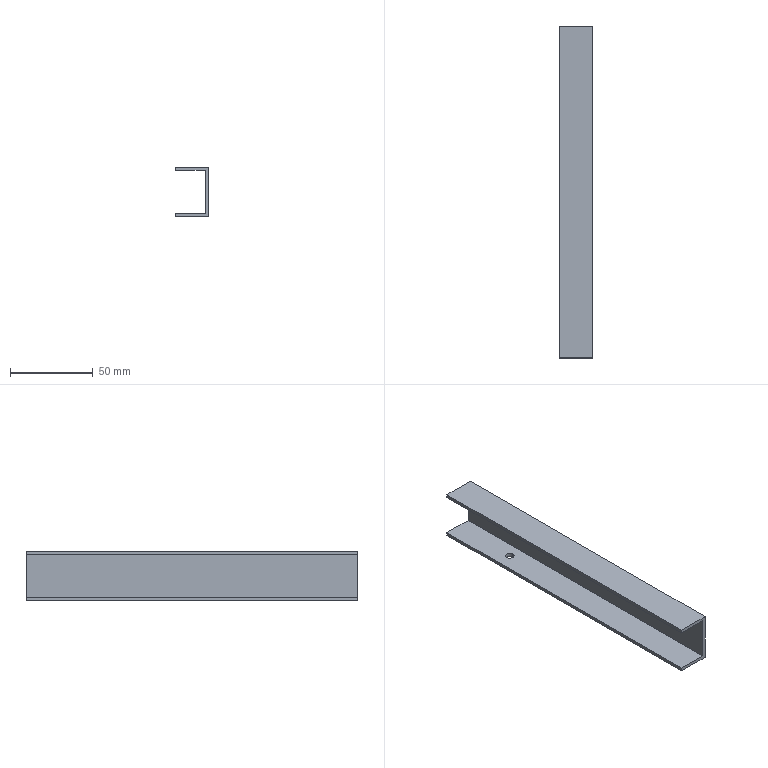Component | SolidWorks | Copy_of_Copy_of_Part4-1 | 1 solid | 12 faces | box 20 x 200 x 30 mm | volume 26361 mm3 | plane 10 | cylinder 2 | commonest cylinder face diameters 5 x2
build123d program:
from build123d import *

# Parameters (mm, degrees)
EXTRUDE_THIN1_DEPTH = 200
SKETCH4_R           = 2.5
CUT_EXTRUDE1_DEPTH  = 10


with BuildPart() as part:
    # Sketch2 → Extrude-Thin1 (new body)
    with BuildSketch(Plane(origin=(0, 0, 0), x_dir=(1, 0, 0), z_dir=(0, 1, 0))):
        Polygon((-173.819, 20), (-173.819, 0), (-143.819, 0), (-143.819, 20), (-145.819, 20), (-145.819, 2), (-171.819, 2), (-171.819, 20), align=None)
    extrude(amount=EXTRUDE_THIN1_DEPTH)

    # Sketch4 → Cut-Extrude1 (cut)
    with BuildSketch(Plane(origin=(-143.819, 0, 0), x_dir=(0, 0, -1), z_dir=(1, 0, 0))):
        with Locations((10.231, 156.085)):
            Circle(SKETCH4_R)
    extrude(amount=-CUT_EXTRUDE1_DEPTH, mode=Mode.SUBTRACT)


solid = part.part

# Placed as in the assembly
solid = solid.moved(Location((152, 30, -459.911), (0, 90, 0)))
STEP:
#1=CARTESIAN_POINT('',(5.68,7.326,-12.366));
#2=VERTEX_POINT('',#1);
#3=CARTESIAN_POINT('',(5.483,7.326,-12.366));
#4=VERTEX_POINT('',#3);
#5=CARTESIAN_POINT('',(5.581,7.326,-12.366));
#6=DIRECTION('',(0.,0.,-1.));
#7=DIRECTION('',(-1.,0.,0.));
#8=AXIS2_PLACEMENT_3D('',#5,#6,#7);
#9=CIRCLE('',#8,0.09843);
#10=EDGE_CURVE('',#2,#4,#9,.T.);
#11=ORIENTED_EDGE('',*,*,#10,.F.);
#12=CARTESIAN_POINT('',(5.68,7.326,-12.445));
#13=VERTEX_POINT('',#12);
#14=CARTESIAN_POINT('',(5.68,7.326,-12.051));
#15=DIRECTION('',(0.,0.,-1.));
#16=VECTOR('',#15,39.37);
#17=LINE('',#14,#16);
#18=EDGE_CURVE('',#2,#13,#17,.T.);
#19=ORIENTED_EDGE('',*,*,#18,.T.);
#20=CARTESIAN_POINT('',(5.483,7.326,-12.445));
#21=VERTEX_POINT('',#20);
#22=CARTESIAN_POINT('',(5.581,7.326,-12.445));
#23=DIRECTION('',(0.,0.,-1.));
#24=DIRECTION('',(-1.,0.,0.));
#25=AXIS2_PLACEMENT_3D('',#22,#23,#24);
#26=CIRCLE('',#25,0.09843);
#27=EDGE_CURVE('',#13,#21,#26,.T.);
#28=ORIENTED_EDGE('',*,*,#27,.T.);
#29=CARTESIAN_POINT('',(5.483,7.326,-12.051));
#30=DIRECTION('',(0.,0.,-1.));
#31=VECTOR('',#30,39.37);
#32=LINE('',#29,#31);
#33=EDGE_CURVE('',#4,#21,#32,.T.);
#34=ORIENTED_EDGE('',*,*,#33,.F.);
#35=EDGE_LOOP('',(#11,#19,#28,#34));
#36=FACE_OUTER_BOUND('',#35,.T.);
#37=CARTESIAN_POINT('',(5.581,7.326,-12.051));
#38=DIRECTION('',(0.,0.,-1.));
#39=DIRECTION('',(-1.,0.,0.));
#40=AXIS2_PLACEMENT_3D('',#37,#38,#39);
#41=CYLINDRICAL_SURFACE('',#40,0.09843);
#42=ADVANCED_FACE('',(#36),#41,.F.);
#43=CARTESIAN_POINT('',(5.906,1.181,-11.342));
#44=VERTEX_POINT('',#43);
#45=CARTESIAN_POINT('',(5.197,1.181,-11.342));
#46=VERTEX_POINT('',#45);
#47=CARTESIAN_POINT('',(5.197,1.181,-11.342));
#48=DIRECTION('',(-1.,0.,0.));
#49=VECTOR('',#48,39.37);
#50=LINE('',#47,#49);
#51=EDGE_CURVE('',#44,#46,#50,.T.);
#52=ORIENTED_EDGE('',*,*,#51,.T.);
#53=CARTESIAN_POINT('',(5.197,9.055,-11.342));
#54=VERTEX_POINT('',#53);
#55=CARTESIAN_POINT('',(5.197,9.055,-11.342));
#56=DIRECTION('',(0.,-1.,0.));
#57=VECTOR('',#56,39.37);
#58=LINE('',#55,#57);
#59=EDGE_CURVE('',#54,#46,#58,.T.);
#60=ORIENTED_EDGE('',*,*,#59,.F.);
#61=CARTESIAN_POINT('',(5.906,9.055,-11.342));
#62=VERTEX_POINT('',#61);
#63=CARTESIAN_POINT('',(5.197,9.055,-11.342));
#64=DIRECTION('',(-1.,0.,0.));
#65=VECTOR('',#64,39.37);
#66=LINE('',#63,#65);
#67=EDGE_CURVE('',#62,#54,#66,.T.);
#68=ORIENTED_EDGE('',*,*,#67,.F.);
#69=CARTESIAN_POINT('',(5.906,9.055,-11.342));
#70=DIRECTION('',(0.,-1.,0.));
#71=VECTOR('',#70,39.37);
#72=LINE('',#69,#71);
#73=EDGE_CURVE('',#62,#44,#72,.T.);
#74=ORIENTED_EDGE('',*,*,#73,.T.);
#75=EDGE_LOOP('',(#52,#60,#68,#74));
#76=FACE_OUTER_BOUND('',#75,.T.);
#77=CARTESIAN_POINT('',(5.197,9.055,-11.342));
#78=DIRECTION('',(0.,0.,1.));
#79=DIRECTION('',(1.,0.,0.));
#80=AXIS2_PLACEMENT_3D('',#77,#78,#79);
#81=PLANE('',#80);
#82=ADVANCED_FACE('',(#76),#81,.F.);
#83=CARTESIAN_POINT('',(5.197,1.181,-11.263));
#84=VERTEX_POINT('',#83);
#85=CARTESIAN_POINT('',(5.197,1.181,-11.263));
#86=DIRECTION('',(0.,0.,-1.));
#87=VECTOR('',#86,39.37);
#88=LINE('',#85,#87);
#89=EDGE_CURVE('',#84,#46,#88,.T.);
#90=ORIENTED_EDGE('',*,*,#89,.F.);
#91=CARTESIAN_POINT('',(5.197,9.055,-11.263));
#92=VERTEX_POINT('',#91);
#93=CARTESIAN_POINT('',(5.197,9.055,-11.263));
#94=DIRECTION('',(0.,-1.,0.));
#95=VECTOR('',#94,39.37);
#96=LINE('',#93,#95);
#97=EDGE_CURVE('',#92,#84,#96,.T.);
#98=ORIENTED_EDGE('',*,*,#97,.F.);
#99=CARTESIAN_POINT('',(5.197,9.055,-11.263));
#100=DIRECTION('',(0.,0.,-1.));
#101=VECTOR('',#100,39.37);
#102=LINE('',#99,#101);
#103=EDGE_CURVE('',#92,#54,#102,.T.);
#104=ORIENTED_EDGE('',*,*,#103,.T.);
#105=ORIENTED_EDGE('',*,*,#59,.T.);
#106=EDGE_LOOP('',(#90,#98,#104,#105));
#107=FACE_OUTER_BOUND('',#106,.T.);
#108=CARTESIAN_POINT('',(5.197,9.055,-11.263));
#109=DIRECTION('',(-1.,0.,0.));
#110=DIRECTION('',(0.,0.,1.));
#111=AXIS2_PLACEMENT_3D('',#108,#109,#110);
#112=PLANE('',#111);
#113=ADVANCED_FACE('',(#107),#112,.T.);
#114=CARTESIAN_POINT('',(5.984,1.181,-11.263));
#115=VERTEX_POINT('',#114);
#116=CARTESIAN_POINT('',(5.197,1.181,-11.263));
#117=DIRECTION('',(-1.,0.,0.));
#118=VECTOR('',#117,39.37);
#119=LINE('',#116,#118);
#120=EDGE_CURVE('',#115,#84,#119,.T.);
#121=ORIENTED_EDGE('',*,*,#120,.F.);
#122=CARTESIAN_POINT('',(5.984,9.055,-11.263));
#123=VERTEX_POINT('',#122);
#124=CARTESIAN_POINT('',(5.984,9.055,-11.263));
#125=DIRECTION('',(0.,-1.,0.));
#126=VECTOR('',#125,39.37);
#127=LINE('',#124,#126);
#128=EDGE_CURVE('',#123,#115,#127,.T.);
#129=ORIENTED_EDGE('',*,*,#128,.F.);
#130=CARTESIAN_POINT('',(5.197,9.055,-11.263));
#131=DIRECTION('',(-1.,0.,0.));
#132=VECTOR('',#131,39.37);
#133=LINE('',#130,#132);
#134=EDGE_CURVE('',#123,#92,#133,.T.);
#135=ORIENTED_EDGE('',*,*,#134,.T.);
#136=ORIENTED_EDGE('',*,*,#97,.T.);
#137=EDGE_LOOP('',(#121,#129,#135,#136));
#138=FACE_OUTER_BOUND('',#137,.T.);
#139=CARTESIAN_POINT('',(5.197,9.055,-11.263));
#140=DIRECTION('',(0.,0.,1.));
#141=DIRECTION('',(1.,0.,0.));
#142=AXIS2_PLACEMENT_3D('',#139,#140,#141);
#143=PLANE('',#142);
#144=ADVANCED_FACE('',(#138),#143,.T.);
#145=CARTESIAN_POINT('',(5.984,1.181,-12.445));
#146=VERTEX_POINT('',#145);
#147=CARTESIAN_POINT('',(5.984,1.181,-11.263));
#148=DIRECTION('',(0.,0.,1.));
#149=VECTOR('',#148,39.37);
#150=LINE('',#147,#149);
#151=EDGE_CURVE('',#146,#115,#150,.T.);
#152=ORIENTED_EDGE('',*,*,#151,.F.);
#153=CARTESIAN_POINT('',(5.984,9.055,-12.445));
#154=VERTEX_POINT('',#153);
#155=CARTESIAN_POINT('',(5.984,9.055,-12.445));
#156=DIRECTION('',(0.,-1.,0.));
#157=VECTOR('',#156,39.37);
#158=LINE('',#155,#157);
#159=EDGE_CURVE('',#154,#146,#158,.T.);
#160=ORIENTED_EDGE('',*,*,#159,.F.);
#161=CARTESIAN_POINT('',(5.984,9.055,-11.263));
#162=DIRECTION('',(0.,0.,1.));
#163=VECTOR('',#162,39.37);
#164=LINE('',#161,#163);
#165=EDGE_CURVE('',#154,#123,#164,.T.);
#166=ORIENTED_EDGE('',*,*,#165,.T.);
#167=ORIENTED_EDGE('',*,*,#128,.T.);
#168=EDGE_LOOP('',(#152,#160,#166,#167));
#169=FACE_OUTER_BOUND('',#168,.T.);
#170=CARTESIAN_POINT('',(5.984,9.055,-11.263));
#171=DIRECTION('',(1.,0.,0.));
#172=DIRECTION('',(0.,0.,-1.));
#173=AXIS2_PLACEMENT_3D('',#170,#171,#172);
#174=PLANE('',#173);
#175=ADVANCED_FACE('',(#169),#174,.T.);
#176=CARTESIAN_POINT('',(5.581,7.326,-12.445));
#177=DIRECTION('',(0.,0.,-1.));
#178=DIRECTION('',(-1.,0.,0.));
#179=AXIS2_PLACEMENT_3D('',#176,#177,#178);
#180=CIRCLE('',#179,0.09843);
#181=EDGE_CURVE('',#21,#13,#180,.T.);
#182=ORIENTED_EDGE('',*,*,#181,.F.);
#183=ORIENTED_EDGE('',*,*,#27,.F.);
#184=EDGE_LOOP('',(#182,#183));
#185=FACE_BOUND('',#184,.T.);
#186=CARTESIAN_POINT('',(5.197,1.181,-12.445));
#187=VERTEX_POINT('',#186);
#188=CARTESIAN_POINT('',(5.197,1.181,-12.445));
#189=DIRECTION('',(1.,0.,0.));
#190=VECTOR('',#189,39.37);
#191=LINE('',#188,#190);
#192=EDGE_CURVE('',#187,#146,#191,.T.);
#193=ORIENTED_EDGE('',*,*,#192,.F.);
#194=CARTESIAN_POINT('',(5.197,9.055,-12.445));
#195=VERTEX_POINT('',#194);
#196=CARTESIAN_POINT('',(5.197,9.055,-12.445));
#197=DIRECTION('',(0.,-1.,0.));
#198=VECTOR('',#197,39.37);
#199=LINE('',#196,#198);
#200=EDGE_CURVE('',#195,#187,#199,.T.);
#201=ORIENTED_EDGE('',*,*,#200,.F.);
#202=CARTESIAN_POINT('',(5.197,9.055,-12.445));
#203=DIRECTION('',(1.,0.,0.));
#204=VECTOR('',#203,39.37);
#205=LINE('',#202,#204);
#206=EDGE_CURVE('',#195,#154,#205,.T.);
#207=ORIENTED_EDGE('',*,*,#206,.T.);
#208=ORIENTED_EDGE('',*,*,#159,.T.);
#209=EDGE_LOOP('',(#193,#201,#207,#208));
#210=FACE_OUTER_BOUND('',#209,.T.);
#211=CARTESIAN_POINT('',(5.197,9.055,-12.445));
#212=DIRECTION('',(0.,0.,-1.));
#213=DIRECTION('',(-1.,0.,0.));
#214=AXIS2_PLACEMENT_3D('',#211,#212,#213);
#215=PLANE('',#214);
#216=ADVANCED_FACE('',(#185,#210),#215,.T.);
#217=CARTESIAN_POINT('',(5.197,1.181,-12.366));
#218=VERTEX_POINT('',#217);
#219=CARTESIAN_POINT('',(5.197,1.181,-12.366));
#220=DIRECTION('',(0.,0.,-1.));
#221=VECTOR('',#220,39.37);
#222=LINE('',#219,#221);
#223=EDGE_CURVE('',#218,#187,#222,.T.);
#224=ORIENTED_EDGE('',*,*,#223,.F.);
#225=CARTESIAN_POINT('',(5.197,9.055,-12.366));
#226=VERTEX_POINT('',#225);
#227=CARTESIAN_POINT('',(5.197,9.055,-12.366));
#228=DIRECTION('',(0.,-1.,0.));
#229=VECTOR('',#228,39.37);
#230=LINE('',#227,#229);
#231=EDGE_CURVE('',#226,#218,#230,.T.);
#232=ORIENTED_EDGE('',*,*,#231,.F.);
#233=CARTESIAN_POINT('',(5.197,9.055,-12.366));
#234=DIRECTION('',(0.,0.,-1.));
#235=VECTOR('',#234,39.37);
#236=LINE('',#233,#235);
#237=EDGE_CURVE('',#226,#195,#236,.T.);
#238=ORIENTED_EDGE('',*,*,#237,.T.);
#239=ORIENTED_EDGE('',*,*,#200,.T.);
#240=EDGE_LOOP('',(#224,#232,#238,#239));
#241=FACE_OUTER_BOUND('',#240,.T.);
#242=CARTESIAN_POINT('',(5.197,9.055,-12.366));
#243=DIRECTION('',(-1.,0.,0.));
#244=DIRECTION('',(0.,0.,1.));
#245=AXIS2_PLACEMENT_3D('',#242,#243,#244);
#246=PLANE('',#245);
#247=ADVANCED_FACE('',(#241),#246,.T.);
#248=CARTESIAN_POINT('',(5.581,7.326,-12.366));
#249=DIRECTION('',(0.,0.,-1.));
#250=DIRECTION('',(-1.,0.,0.));
#251=AXIS2_PLACEMENT_3D('',#248,#249,#250);
#252=CIRCLE('',#251,0.09843);
#253=EDGE_CURVE('',#4,#2,#252,.T.);
#254=ORIENTED_EDGE('',*,*,#253,.T.);
#255=ORIENTED_EDGE('',*,*,#10,.T.);
#256=EDGE_LOOP('',(#254,#255));
#257=FACE_BOUND('',#256,.T.);
#258=CARTESIAN_POINT('',(5.906,1.181,-12.366));
#259=VERTEX_POINT('',#258);
#260=CARTESIAN_POINT('',(5.197,1.181,-12.366));
#261=DIRECTION('',(1.,0.,0.));
#262=VECTOR('',#261,39.37);
#263=LINE('',#260,#262);
#264=EDGE_CURVE('',#218,#259,#263,.T.);
#265=ORIENTED_EDGE('',*,*,#264,.T.);
#266=CARTESIAN_POINT('',(5.906,9.055,-12.366));
#267=VERTEX_POINT('',#266);
#268=CARTESIAN_POINT('',(5.906,9.055,-12.366));
#269=DIRECTION('',(0.,-1.,0.));
#270=VECTOR('',#269,39.37);
#271=LINE('',#268,#270);
#272=EDGE_CURVE('',#267,#259,#271,.T.);
#273=ORIENTED_EDGE('',*,*,#272,.F.);
#274=CARTESIAN_POINT('',(5.197,9.055,-12.366));
#275=DIRECTION('',(1.,0.,0.));
#276=VECTOR('',#275,39.37);
#277=LINE('',#274,#276);
#278=EDGE_CURVE('',#226,#267,#277,.T.);
#279=ORIENTED_EDGE('',*,*,#278,.F.);
#280=ORIENTED_EDGE('',*,*,#231,.T.);
#281=EDGE_LOOP('',(#265,#273,#279,#280));
#282=FACE_OUTER_BOUND('',#281,.T.);
#283=CARTESIAN_POINT('',(5.197,9.055,-12.366));
#284=DIRECTION('',(0.,0.,-1.));
#285=DIRECTION('',(-1.,0.,0.));
#286=AXIS2_PLACEMENT_3D('',#283,#284,#285);
#287=PLANE('',#286);
#288=ADVANCED_FACE('',(#257,#282),#287,.F.);
#289=CARTESIAN_POINT('',(5.906,1.181,-11.263));
#290=DIRECTION('',(0.,0.,1.));
#291=VECTOR('',#290,39.37);
#292=LINE('',#289,#291);
#293=EDGE_CURVE('',#259,#44,#292,.T.);
#294=ORIENTED_EDGE('',*,*,#293,.T.);
#295=ORIENTED_EDGE('',*,*,#73,.F.);
#296=CARTESIAN_POINT('',(5.906,9.055,-11.263));
#297=DIRECTION('',(0.,0.,1.));
#298=VECTOR('',#297,39.37);
#299=LINE('',#296,#298);
#300=EDGE_CURVE('',#267,#62,#299,.T.);
#301=ORIENTED_EDGE('',*,*,#300,.F.);
#302=ORIENTED_EDGE('',*,*,#272,.T.);
#303=EDGE_LOOP('',(#294,#295,#301,#302));
#304=FACE_OUTER_BOUND('',#303,.T.);
#305=CARTESIAN_POINT('',(5.906,9.055,-11.263));
#306=DIRECTION('',(1.,0.,0.));
#307=DIRECTION('',(0.,0.,-1.));
#308=AXIS2_PLACEMENT_3D('',#305,#306,#307);
#309=PLANE('',#308);
#310=ADVANCED_FACE('',(#304),#309,.F.);
#311=ORIENTED_EDGE('',*,*,#67,.T.);
#312=ORIENTED_EDGE('',*,*,#103,.F.);
#313=ORIENTED_EDGE('',*,*,#134,.F.);
#314=ORIENTED_EDGE('',*,*,#165,.F.);
#315=ORIENTED_EDGE('',*,*,#206,.F.);
#316=ORIENTED_EDGE('',*,*,#237,.F.);
#317=ORIENTED_EDGE('',*,*,#278,.T.);
#318=ORIENTED_EDGE('',*,*,#300,.T.);
#319=EDGE_LOOP('',(#311,#312,#313,#314,#315,#316,#317,#318));
#320=FACE_OUTER_BOUND('',#319,.T.);
#321=CARTESIAN_POINT('',(5.984,9.055,-18.107));
#322=DIRECTION('',(0.,-1.,0.));
#323=DIRECTION('',(0.,0.,1.));
#324=AXIS2_PLACEMENT_3D('',#321,#322,#323);
#325=PLANE('',#324);
#326=ADVANCED_FACE('',(#320),#325,.F.);
#327=ORIENTED_EDGE('',*,*,#51,.F.);
#328=ORIENTED_EDGE('',*,*,#293,.F.);
#329=ORIENTED_EDGE('',*,*,#264,.F.);
#330=ORIENTED_EDGE('',*,*,#223,.T.);
#331=ORIENTED_EDGE('',*,*,#192,.T.);
#332=ORIENTED_EDGE('',*,*,#151,.T.);
#333=ORIENTED_EDGE('',*,*,#120,.T.);
#334=ORIENTED_EDGE('',*,*,#89,.T.);
#335=EDGE_LOOP('',(#327,#328,#329,#330,#331,#332,#333,#334));
#336=FACE_OUTER_BOUND('',#335,.T.);
#337=CARTESIAN_POINT('',(5.984,1.181,-18.107));
#338=DIRECTION('',(0.,-1.,0.));
#339=DIRECTION('',(0.,0.,1.));
#340=AXIS2_PLACEMENT_3D('',#337,#338,#339);
#341=PLANE('',#340);
#342=ADVANCED_FACE('',(#336),#341,.T.);
#343=ORIENTED_EDGE('',*,*,#18,.F.);
#344=ORIENTED_EDGE('',*,*,#253,.F.);
#345=ORIENTED_EDGE('',*,*,#33,.T.);
#346=ORIENTED_EDGE('',*,*,#181,.T.);
#347=EDGE_LOOP('',(#343,#344,#345,#346));
#348=FACE_OUTER_BOUND('',#347,.T.);
#349=CARTESIAN_POINT('',(5.581,7.326,-12.051));
#350=DIRECTION('',(0.,0.,-1.));
#351=DIRECTION('',(-1.,0.,0.));
#352=AXIS2_PLACEMENT_3D('',#349,#350,#351);
#353=CYLINDRICAL_SURFACE('',#352,0.09843);
#354=ADVANCED_FACE('',(#348),#353,.F.);
#355=CLOSED_SHELL('',(#42,#82,#113,#144,#175,#216,#247,#288,#310,#326,#342,#354));
#356=MANIFOLD_SOLID_BREP('',#355);
#357=CARTESIAN_POINT('',(0.,0.,0.));
#358=DIRECTION('',(0.,0.,1.));
#359=DIRECTION('',(1.,0.,0.));
#360=AXIS2_PLACEMENT_3D('',#357,#358,#359);
#361=(LENGTH_UNIT()NAMED_UNIT(*)SI_UNIT($,.METRE.));
#362=LENGTH_MEASURE_WITH_UNIT(LENGTH_MEASURE(0.0254),#361);
#363=DIMENSIONAL_EXPONENTS(1.,0.,0.,0.,0.,0.,0.);
#364=(CONVERSION_BASED_UNIT('',#362)LENGTH_UNIT()NAMED_UNIT(#363));
#365=UNCERTAINTY_MEASURE_WITH_UNIT(LENGTH_MEASURE(0.00001),#364,'','');
#366=(NAMED_UNIT(*)PLANE_ANGLE_UNIT()SI_UNIT($,.RADIAN.));
#367=(NAMED_UNIT(*)SI_UNIT($,.STERADIAN.)SOLID_ANGLE_UNIT());
#368=(GEOMETRIC_REPRESENTATION_CONTEXT(3)GLOBAL_UNCERTAINTY_ASSIGNED_CONTEXT((#365))GLOBAL_UNIT_ASSIGNED_CONTEXT((#364,#366,#367))REPRESENTATION_CONTEXT('',''));
#369=ADVANCED_BREP_SHAPE_REPRESENTATION('',(#356,#360),#368);
#370=COLOUR_RGB('',0.7922,0.8196,0.9333);
#371=FILL_AREA_STYLE_COLOUR('',#370);
#372=FILL_AREA_STYLE('',(#371));
#373=SURFACE_STYLE_FILL_AREA(#372);
#374=SURFACE_SIDE_STYLE('',(#373));
#375=SURFACE_STYLE_USAGE(.BOTH.,#374);
#376=PRESENTATION_STYLE_ASSIGNMENT((#375));
#377=STYLED_ITEM('',(#376),#356);
#378=(LENGTH_UNIT()NAMED_UNIT(*)SI_UNIT($,.METRE.));
#379=LENGTH_MEASURE_WITH_UNIT(LENGTH_MEASURE(0.0254),#378);
#380=DIMENSIONAL_EXPONENTS(1.,0.,0.,0.,0.,0.,0.);
#381=(CONVERSION_BASED_UNIT('',#379)LENGTH_UNIT()NAMED_UNIT(#380));
#382=UNCERTAINTY_MEASURE_WITH_UNIT(LENGTH_MEASURE(0.00001),#381,'','');
#383=(NAMED_UNIT(*)PLANE_ANGLE_UNIT()SI_UNIT($,.RADIAN.));
#384=(NAMED_UNIT(*)SI_UNIT($,.STERADIAN.)SOLID_ANGLE_UNIT());
#385=(GEOMETRIC_REPRESENTATION_CONTEXT(3)GLOBAL_UNCERTAINTY_ASSIGNED_CONTEXT((#382))GLOBAL_UNIT_ASSIGNED_CONTEXT((#381,#383,#384))REPRESENTATION_CONTEXT('',''));
#386=MECHANICAL_DESIGN_GEOMETRIC_PRESENTATION_REPRESENTATION('',(#377),#385);
#387=PRESENTATION_LAYER_ASSIGNMENT('','',(#377));